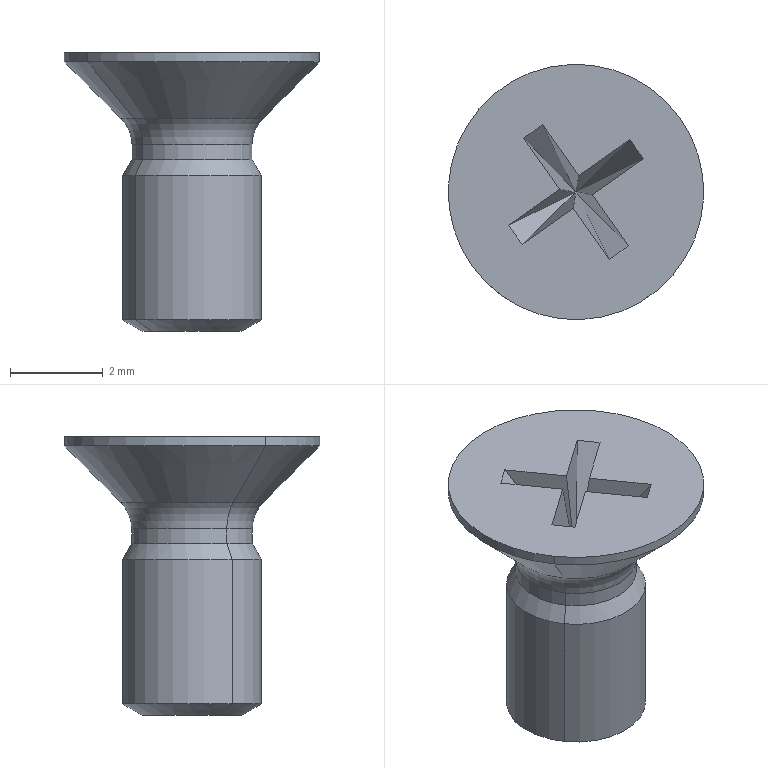Component | SolidWorks | MGL-PACK-03-00Fixture-1_PhillipsCountersunkScrewM3_6[GB_T819.1-2000]-1 | 1 solid | 28 faces | box 5.5 x 5.5 x 6 mm | volume 51 mm3 | plane 14 | cone 6 | cylinder 6 | torus 2 | commonest cylinder face diameters 3 x2 2.598 x2 5.5 x2
STEP:
#1=COLOUR_RGB('',0.7922,0.8196,0.9333);
#2=FILL_AREA_STYLE_COLOUR('',#1);
#3=FILL_AREA_STYLE('',(#2));
#4=SURFACE_STYLE_FILL_AREA(#3);
#5=SURFACE_SIDE_STYLE('',(#4));
#6=SURFACE_STYLE_USAGE(.BOTH.,#5);
#7=PRESENTATION_STYLE_ASSIGNMENT((#6));
#8=CARTESIAN_POINT('',(10.566,1.343,-10.524));
#9=VERTEX_POINT('',#8);
#10=CARTESIAN_POINT('',(10.497,1.295,-10.524));
#11=VERTEX_POINT('',#10);
#12=CARTESIAN_POINT('',(10.531,1.319,-10.524));
#13=DIRECTION('',(-0.,0.,-1.));
#14=DIRECTION('',(0.8166,0.5772,0.));
#15=AXIS2_PLACEMENT_3D('',#12,#13,#14);
#16=CIRCLE('',#15,0.04201);
#17=EDGE_CURVE('',#9,#11,#16,.T.);
#18=ORIENTED_EDGE('',*,*,#17,.F.);
#19=CARTESIAN_POINT('',(10.58,1.353,-10.514));
#20=VERTEX_POINT('',#19);
#21=CARTESIAN_POINT('',(10.58,1.353,-10.514));
#22=DIRECTION('',(0.7091,0.5012,0.4959));
#23=VECTOR('',#22,39.37);
#24=LINE('',#21,#23);
#25=EDGE_CURVE('',#9,#20,#24,.T.);
#26=ORIENTED_EDGE('',*,*,#25,.T.);
#27=CARTESIAN_POINT('',(10.483,1.285,-10.514));
#28=VERTEX_POINT('',#27);
#29=CARTESIAN_POINT('',(10.531,1.319,-10.514));
#30=DIRECTION('',(-0.,0.,-1.));
#31=DIRECTION('',(0.8166,0.5772,0.));
#32=AXIS2_PLACEMENT_3D('',#29,#30,#31);
#33=CIRCLE('',#32,0.05906);
#34=EDGE_CURVE('',#20,#28,#33,.T.);
#35=ORIENTED_EDGE('',*,*,#34,.T.);
#36=CARTESIAN_POINT('',(10.483,1.285,-10.514));
#37=DIRECTION('',(-0.7091,-0.5012,0.4959));
#38=VECTOR('',#37,39.37);
#39=LINE('',#36,#38);
#40=EDGE_CURVE('',#11,#28,#39,.T.);
#41=ORIENTED_EDGE('',*,*,#40,.F.);
#42=EDGE_LOOP('',(#18,#26,#35,#41));
#43=FACE_OUTER_BOUND('',#42,.T.);
#44=CARTESIAN_POINT('',(10.531,1.319,-10.514));
#45=DIRECTION('',(0.,-0.,1.));
#46=DIRECTION('',(-0.8166,-0.5772,0.));
#47=AXIS2_PLACEMENT_3D('',#44,#45,#46);
#48=CONICAL_SURFACE('',#47,0.05906,1.052);
#49=ADVANCED_FACE('',(#43),#48,.T.);
#50=ORIENTED_EDGE('',*,*,#34,.F.);
#51=CARTESIAN_POINT('',(10.58,1.353,-10.392));
#52=VERTEX_POINT('',#51);
#53=CARTESIAN_POINT('',(10.58,1.353,-10.287));
#54=DIRECTION('',(0.,-0.,1.));
#55=VECTOR('',#54,39.37);
#56=LINE('',#53,#55);
#57=EDGE_CURVE('',#20,#52,#56,.T.);
#58=ORIENTED_EDGE('',*,*,#57,.T.);
#59=CARTESIAN_POINT('',(10.483,1.285,-10.392));
#60=VERTEX_POINT('',#59);
#61=CARTESIAN_POINT('',(10.531,1.319,-10.392));
#62=DIRECTION('',(0.,-0.,1.));
#63=DIRECTION('',(-0.8166,-0.5772,0.));
#64=AXIS2_PLACEMENT_3D('',#61,#62,#63);
#65=CIRCLE('',#64,0.05906);
#66=EDGE_CURVE('',#60,#52,#65,.T.);
#67=ORIENTED_EDGE('',*,*,#66,.F.);
#68=CARTESIAN_POINT('',(10.483,1.285,-10.287));
#69=DIRECTION('',(0.,-0.,1.));
#70=VECTOR('',#69,39.37);
#71=LINE('',#68,#70);
#72=EDGE_CURVE('',#28,#60,#71,.T.);
#73=ORIENTED_EDGE('',*,*,#72,.F.);
#74=EDGE_LOOP('',(#50,#58,#67,#73));
#75=FACE_OUTER_BOUND('',#74,.T.);
#76=CARTESIAN_POINT('',(10.531,1.319,-10.287));
#77=DIRECTION('',(0.,-0.,1.));
#78=DIRECTION('',(-0.8166,-0.5772,0.));
#79=AXIS2_PLACEMENT_3D('',#76,#77,#78);
#80=CYLINDRICAL_SURFACE('',#79,0.05906);
#81=ADVANCED_FACE('',(#75),#80,.T.);
#82=CARTESIAN_POINT('',(10.49,1.289,-10.378));
#83=VERTEX_POINT('',#82);
#84=CARTESIAN_POINT('',(10.573,1.348,-10.378));
#85=VERTEX_POINT('',#84);
#86=CARTESIAN_POINT('',(10.531,1.319,-10.378));
#87=DIRECTION('',(0.,-0.,1.));
#88=DIRECTION('',(-0.8166,-0.5772,0.));
#89=AXIS2_PLACEMENT_3D('',#86,#87,#88);
#90=CIRCLE('',#89,0.05114);
#91=EDGE_CURVE('',#83,#85,#90,.T.);
#92=ORIENTED_EDGE('',*,*,#91,.F.);
#93=CARTESIAN_POINT('',(10.483,1.285,-10.392));
#94=DIRECTION('',(-0.4083,-0.2886,-0.866));
#95=VECTOR('',#94,39.37);
#96=LINE('',#93,#95);
#97=EDGE_CURVE('',#83,#60,#96,.T.);
#98=ORIENTED_EDGE('',*,*,#97,.T.);
#99=ORIENTED_EDGE('',*,*,#66,.T.);
#100=CARTESIAN_POINT('',(10.58,1.353,-10.392));
#101=DIRECTION('',(0.4083,0.2886,-0.866));
#102=VECTOR('',#101,39.37);
#103=LINE('',#100,#102);
#104=EDGE_CURVE('',#85,#52,#103,.T.);
#105=ORIENTED_EDGE('',*,*,#104,.F.);
#106=EDGE_LOOP('',(#92,#98,#99,#105));
#107=FACE_OUTER_BOUND('',#106,.T.);
#108=CARTESIAN_POINT('',(10.531,1.319,-10.392));
#109=DIRECTION('',(-0.,0.,-1.));
#110=DIRECTION('',(0.8166,0.5772,0.));
#111=AXIS2_PLACEMENT_3D('',#108,#109,#110);
#112=CONICAL_SURFACE('',#111,0.05906,0.5236);
#113=ADVANCED_FACE('',(#107),#112,.T.);
#114=ORIENTED_EDGE('',*,*,#91,.T.);
#115=CARTESIAN_POINT('',(10.573,1.348,-10.365));
#116=VERTEX_POINT('',#115);
#117=CARTESIAN_POINT('',(10.573,1.348,-10.287));
#118=DIRECTION('',(0.,-0.,1.));
#119=VECTOR('',#118,39.37);
#120=LINE('',#117,#119);
#121=EDGE_CURVE('',#85,#116,#120,.T.);
#122=ORIENTED_EDGE('',*,*,#121,.T.);
#123=CARTESIAN_POINT('',(10.49,1.289,-10.365));
#124=VERTEX_POINT('',#123);
#125=CARTESIAN_POINT('',(10.531,1.319,-10.365));
#126=DIRECTION('',(0.,-0.,1.));
#127=DIRECTION('',(-0.8166,-0.5772,0.));
#128=AXIS2_PLACEMENT_3D('',#125,#126,#127);
#129=CIRCLE('',#128,0.05114);
#130=EDGE_CURVE('',#124,#116,#129,.T.);
#131=ORIENTED_EDGE('',*,*,#130,.F.);
#132=CARTESIAN_POINT('',(10.49,1.289,-10.287));
#133=DIRECTION('',(0.,-0.,1.));
#134=VECTOR('',#133,39.37);
#135=LINE('',#132,#134);
#136=EDGE_CURVE('',#83,#124,#135,.T.);
#137=ORIENTED_EDGE('',*,*,#136,.F.);
#138=EDGE_LOOP('',(#114,#122,#131,#137));
#139=FACE_OUTER_BOUND('',#138,.T.);
#140=CARTESIAN_POINT('',(10.531,1.319,-10.287));
#141=DIRECTION('',(0.,-0.,1.));
#142=DIRECTION('',(-0.8166,-0.5772,0.));
#143=AXIS2_PLACEMENT_3D('',#140,#141,#142);
#144=CYLINDRICAL_SURFACE('',#143,0.05114);
#145=ADVANCED_FACE('',(#139),#144,.T.);
#146=CARTESIAN_POINT('',(10.581,1.354,-10.343));
#147=VERTEX_POINT('',#146);
#148=CARTESIAN_POINT('',(10.482,1.284,-10.343));
#149=VERTEX_POINT('',#148);
#150=CARTESIAN_POINT('',(10.531,1.319,-10.343));
#151=DIRECTION('',(0.,-0.,1.));
#152=DIRECTION('',(-0.8166,-0.5772,0.));
#153=AXIS2_PLACEMENT_3D('',#150,#151,#152);
#154=CIRCLE('',#153,0.06037);
#155=EDGE_CURVE('',#147,#149,#154,.T.);
#156=ORIENTED_EDGE('',*,*,#155,.F.);
#157=CARTESIAN_POINT('',(10.599,1.367,-10.365));
#158=DIRECTION('',(0.5772,-0.8166,-0.));
#159=DIRECTION('',(0.8166,0.5772,0.));
#160=AXIS2_PLACEMENT_3D('',#157,#158,#159);
#161=CIRCLE('',#160,0.0315);
#162=EDGE_CURVE('',#147,#116,#161,.T.);
#163=ORIENTED_EDGE('',*,*,#162,.T.);
#164=CARTESIAN_POINT('',(10.531,1.319,-10.365));
#165=DIRECTION('',(0.,-0.,1.));
#166=DIRECTION('',(-0.8166,-0.5772,0.));
#167=AXIS2_PLACEMENT_3D('',#164,#165,#166);
#168=CIRCLE('',#167,0.05114);
#169=EDGE_CURVE('',#116,#124,#168,.T.);
#170=ORIENTED_EDGE('',*,*,#169,.T.);
#171=CARTESIAN_POINT('',(10.464,1.271,-10.365));
#172=DIRECTION('',(-0.5772,0.8166,0.));
#173=DIRECTION('',(-0.8166,-0.5772,0.));
#174=AXIS2_PLACEMENT_3D('',#171,#172,#173);
#175=CIRCLE('',#174,0.0315);
#176=EDGE_CURVE('',#149,#124,#175,.T.);
#177=ORIENTED_EDGE('',*,*,#176,.F.);
#178=EDGE_LOOP('',(#156,#163,#170,#177));
#179=FACE_OUTER_BOUND('',#178,.T.);
#180=CARTESIAN_POINT('',(10.531,1.319,-10.365));
#181=DIRECTION('',(0.,-0.,1.));
#182=DIRECTION('',(-0.8166,-0.5772,-0.));
#183=AXIS2_PLACEMENT_3D('',#180,#181,#182);
#184=TOROIDAL_SURFACE('',#183,0.08264,0.0315);
#185=ADVANCED_FACE('',(#179),#184,.F.);
#186=CARTESIAN_POINT('',(10.531,1.319,-10.343));
#187=DIRECTION('',(0.,-0.,1.));
#188=DIRECTION('',(-0.8166,-0.5772,0.));
#189=AXIS2_PLACEMENT_3D('',#186,#187,#188);
#190=CIRCLE('',#189,0.06037);
#191=EDGE_CURVE('',#149,#147,#190,.T.);
#192=ORIENTED_EDGE('',*,*,#191,.T.);
#193=CARTESIAN_POINT('',(10.62,1.381,-10.295));
#194=VERTEX_POINT('',#193);
#195=CARTESIAN_POINT('',(10.581,1.354,-10.343));
#196=DIRECTION('',(0.5774,0.4081,0.7071));
#197=VECTOR('',#196,39.37);
#198=LINE('',#195,#197);
#199=EDGE_CURVE('',#147,#194,#198,.T.);
#200=ORIENTED_EDGE('',*,*,#199,.T.);
#201=CARTESIAN_POINT('',(10.443,1.256,-10.295));
#202=VERTEX_POINT('',#201);
#203=CARTESIAN_POINT('',(10.531,1.319,-10.295));
#204=DIRECTION('',(0.,-0.,1.));
#205=DIRECTION('',(-0.8166,-0.5772,0.));
#206=AXIS2_PLACEMENT_3D('',#203,#204,#205);
#207=CIRCLE('',#206,0.1083);
#208=EDGE_CURVE('',#202,#194,#207,.T.);
#209=ORIENTED_EDGE('',*,*,#208,.F.);
#210=CARTESIAN_POINT('',(10.482,1.284,-10.343));
#211=DIRECTION('',(-0.5774,-0.4081,0.7071));
#212=VECTOR('',#211,39.37);
#213=LINE('',#210,#212);
#214=EDGE_CURVE('',#149,#202,#213,.T.);
#215=ORIENTED_EDGE('',*,*,#214,.F.);
#216=EDGE_LOOP('',(#192,#200,#209,#215));
#217=FACE_OUTER_BOUND('',#216,.T.);
#218=CARTESIAN_POINT('',(10.531,1.319,-10.343));
#219=DIRECTION('',(0.,-0.,1.));
#220=DIRECTION('',(-0.8166,-0.5772,0.));
#221=AXIS2_PLACEMENT_3D('',#218,#219,#220);
#222=CONICAL_SURFACE('',#221,0.06037,0.7854);
#223=ADVANCED_FACE('',(#217),#222,.T.);
#224=ORIENTED_EDGE('',*,*,#208,.T.);
#225=CARTESIAN_POINT('',(10.62,1.381,-10.287));
#226=VERTEX_POINT('',#225);
#227=CARTESIAN_POINT('',(10.62,1.381,-10.287));
#228=DIRECTION('',(0.,-0.,1.));
#229=VECTOR('',#228,39.37);
#230=LINE('',#227,#229);
#231=EDGE_CURVE('',#194,#226,#230,.T.);
#232=ORIENTED_EDGE('',*,*,#231,.T.);
#233=CARTESIAN_POINT('',(10.443,1.256,-10.287));
#234=VERTEX_POINT('',#233);
#235=CARTESIAN_POINT('',(10.531,1.319,-10.287));
#236=DIRECTION('',(0.,-0.,1.));
#237=DIRECTION('',(-0.8166,-0.5772,0.));
#238=AXIS2_PLACEMENT_3D('',#235,#236,#237);
#239=CIRCLE('',#238,0.1083);
#240=EDGE_CURVE('',#234,#226,#239,.T.);
#241=ORIENTED_EDGE('',*,*,#240,.F.);
#242=CARTESIAN_POINT('',(10.443,1.256,-10.287));
#243=DIRECTION('',(0.,-0.,1.));
#244=VECTOR('',#243,39.37);
#245=LINE('',#242,#244);
#246=EDGE_CURVE('',#202,#234,#245,.T.);
#247=ORIENTED_EDGE('',*,*,#246,.F.);
#248=EDGE_LOOP('',(#224,#232,#241,#247));
#249=FACE_OUTER_BOUND('',#248,.T.);
#250=CARTESIAN_POINT('',(10.531,1.319,-10.287));
#251=DIRECTION('',(0.,-0.,1.));
#252=DIRECTION('',(-0.8166,-0.5772,0.));
#253=AXIS2_PLACEMENT_3D('',#250,#251,#252);
#254=CYLINDRICAL_SURFACE('',#253,0.1083);
#255=ADVANCED_FACE('',(#249),#254,.T.);
#256=ORIENTED_EDGE('',*,*,#240,.T.);
#257=CARTESIAN_POINT('',(10.531,1.319,-10.287));
#258=DIRECTION('',(0.,-0.,1.));
#259=DIRECTION('',(-0.8166,-0.5772,0.));
#260=AXIS2_PLACEMENT_3D('',#257,#258,#259);
#261=CIRCLE('',#260,0.1083);
#262=EDGE_CURVE('',#226,#234,#261,.T.);
#263=ORIENTED_EDGE('',*,*,#262,.T.);
#264=EDGE_LOOP('',(#256,#263));
#265=FACE_OUTER_BOUND('',#264,.T.);
#266=CARTESIAN_POINT('',(10.529,1.305,-10.287));
#267=VERTEX_POINT('',#266);
#268=CARTESIAN_POINT('',(10.56,1.262,-10.287));
#269=VERTEX_POINT('',#268);
#270=CARTESIAN_POINT('',(10.56,1.262,-10.287));
#271=DIRECTION('',(0.5772,-0.8166,-0.));
#272=VECTOR('',#271,39.37);
#273=LINE('',#270,#272);
#274=EDGE_CURVE('',#267,#269,#273,.T.);
#275=ORIENTED_EDGE('',*,*,#274,.F.);
#276=CARTESIAN_POINT('',(10.486,1.275,-10.287));
#277=VERTEX_POINT('',#276);
#278=CARTESIAN_POINT('',(10.589,1.347,-10.287));
#279=DIRECTION('',(0.8166,0.5772,0.));
#280=VECTOR('',#279,39.37);
#281=LINE('',#278,#280);
#282=EDGE_CURVE('',#277,#267,#281,.T.);
#283=ORIENTED_EDGE('',*,*,#282,.F.);
#284=CARTESIAN_POINT('',(10.474,1.291,-10.287));
#285=VERTEX_POINT('',#284);
#286=CARTESIAN_POINT('',(10.486,1.275,-10.287));
#287=DIRECTION('',(0.5772,-0.8166,-0.));
#288=VECTOR('',#287,39.37);
#289=LINE('',#286,#288);
#290=EDGE_CURVE('',#285,#277,#289,.T.);
#291=ORIENTED_EDGE('',*,*,#290,.F.);
#292=CARTESIAN_POINT('',(10.518,1.321,-10.287));
#293=VERTEX_POINT('',#292);
#294=CARTESIAN_POINT('',(10.577,1.363,-10.287));
#295=DIRECTION('',(-0.8166,-0.5772,-0.));
#296=VECTOR('',#295,39.37);
#297=LINE('',#294,#296);
#298=EDGE_CURVE('',#293,#285,#297,.T.);
#299=ORIENTED_EDGE('',*,*,#298,.F.);
#300=CARTESIAN_POINT('',(10.487,1.365,-10.287));
#301=VERTEX_POINT('',#300);
#302=CARTESIAN_POINT('',(10.56,1.262,-10.287));
#303=DIRECTION('',(0.5772,-0.8166,-0.));
#304=VECTOR('',#303,39.37);
#305=LINE('',#302,#304);
#306=EDGE_CURVE('',#301,#293,#305,.T.);
#307=ORIENTED_EDGE('',*,*,#306,.F.);
#308=CARTESIAN_POINT('',(10.503,1.376,-10.287));
#309=VERTEX_POINT('',#308);
#310=CARTESIAN_POINT('',(10.487,1.365,-10.287));
#311=DIRECTION('',(-0.8166,-0.5772,-0.));
#312=VECTOR('',#311,39.37);
#313=LINE('',#310,#312);
#314=EDGE_CURVE('',#309,#301,#313,.T.);
#315=ORIENTED_EDGE('',*,*,#314,.F.);
#316=CARTESIAN_POINT('',(10.534,1.333,-10.287));
#317=VERTEX_POINT('',#316);
#318=CARTESIAN_POINT('',(10.576,1.273,-10.287));
#319=DIRECTION('',(-0.5772,0.8166,0.));
#320=VECTOR('',#319,39.37);
#321=LINE('',#318,#320);
#322=EDGE_CURVE('',#317,#309,#321,.T.);
#323=ORIENTED_EDGE('',*,*,#322,.F.);
#324=CARTESIAN_POINT('',(10.577,1.363,-10.287));
#325=VERTEX_POINT('',#324);
#326=CARTESIAN_POINT('',(10.577,1.363,-10.287));
#327=DIRECTION('',(-0.8166,-0.5772,-0.));
#328=VECTOR('',#327,39.37);
#329=LINE('',#326,#328);
#330=EDGE_CURVE('',#325,#317,#329,.T.);
#331=ORIENTED_EDGE('',*,*,#330,.F.);
#332=CARTESIAN_POINT('',(10.589,1.347,-10.287));
#333=VERTEX_POINT('',#332);
#334=CARTESIAN_POINT('',(10.589,1.347,-10.287));
#335=DIRECTION('',(-0.5772,0.8166,0.));
#336=VECTOR('',#335,39.37);
#337=LINE('',#334,#336);
#338=EDGE_CURVE('',#333,#325,#337,.T.);
#339=ORIENTED_EDGE('',*,*,#338,.F.);
#340=CARTESIAN_POINT('',(10.545,1.317,-10.287));
#341=VERTEX_POINT('',#340);
#342=CARTESIAN_POINT('',(10.589,1.347,-10.287));
#343=DIRECTION('',(0.8166,0.5772,0.));
#344=VECTOR('',#343,39.37);
#345=LINE('',#342,#344);
#346=EDGE_CURVE('',#341,#333,#345,.T.);
#347=ORIENTED_EDGE('',*,*,#346,.F.);
#348=CARTESIAN_POINT('',(10.576,1.273,-10.287));
#349=VERTEX_POINT('',#348);
#350=CARTESIAN_POINT('',(10.576,1.273,-10.287));
#351=DIRECTION('',(-0.5772,0.8166,0.));
#352=VECTOR('',#351,39.37);
#353=LINE('',#350,#352);
#354=EDGE_CURVE('',#349,#341,#353,.T.);
#355=ORIENTED_EDGE('',*,*,#354,.F.);
#356=CARTESIAN_POINT('',(10.56,1.262,-10.287));
#357=DIRECTION('',(0.8166,0.5772,0.));
#358=VECTOR('',#357,39.37);
#359=LINE('',#356,#358);
#360=EDGE_CURVE('',#269,#349,#359,.T.);
#361=ORIENTED_EDGE('',*,*,#360,.F.);
#362=EDGE_LOOP('',(#275,#283,#291,#299,#307,#315,#323,#331,#339,#347,#355,#361));
#363=FACE_BOUND('',#362,.T.);
#364=CARTESIAN_POINT('',(10.531,1.319,-10.287));
#365=DIRECTION('',(-0.,0.,-1.));
#366=DIRECTION('',(0.8166,0.5772,0.));
#367=AXIS2_PLACEMENT_3D('',#364,#365,#366);
#368=PLANE('',#367);
#369=ADVANCED_FACE('',(#265,#363),#368,.F.);
#370=ORIENTED_EDGE('',*,*,#282,.T.);
#371=CARTESIAN_POINT('',(10.531,1.319,-10.37));
#372=VERTEX_POINT('',#371);
#373=CARTESIAN_POINT('',(10.531,1.319,-10.37));
#374=DIRECTION('',(0.02811,0.1636,-0.9861));
#375=VECTOR('',#374,39.37);
#376=LINE('',#373,#375);
#377=EDGE_CURVE('',#267,#372,#376,.T.);
#378=ORIENTED_EDGE('',*,*,#377,.T.);
#379=CARTESIAN_POINT('',(10.486,1.275,-10.287));
#380=DIRECTION('',(0.4383,0.4252,-0.7919));
#381=VECTOR('',#380,39.37);
#382=LINE('',#379,#381);
#383=EDGE_CURVE('',#277,#372,#382,.T.);
#384=ORIENTED_EDGE('',*,*,#383,.F.);
#385=EDGE_LOOP('',(#370,#378,#384));
#386=FACE_OUTER_BOUND('',#385,.T.);
#387=CARTESIAN_POINT('',(10.531,1.319,-10.37));
#388=DIRECTION('',(-0.5731,0.8109,0.1182));
#389=DIRECTION('',(-0.06823,0.09653,-0.993));
#390=AXIS2_PLACEMENT_3D('',#387,#388,#389);
#391=PLANE('',#390);
#392=ADVANCED_FACE('',(#386),#391,.T.);
#393=CARTESIAN_POINT('',(10.589,1.347,-10.287));
#394=DIRECTION('',(-0.5471,-0.2713,-0.7919));
#395=VECTOR('',#394,39.37);
#396=LINE('',#393,#395);
#397=EDGE_CURVE('',#333,#372,#396,.T.);
#398=ORIENTED_EDGE('',*,*,#397,.T.);
#399=CARTESIAN_POINT('',(10.531,1.319,-10.37));
#400=DIRECTION('',(0.1636,-0.02811,0.9861));
#401=VECTOR('',#400,39.37);
#402=LINE('',#399,#401);
#403=EDGE_CURVE('',#372,#341,#402,.T.);
#404=ORIENTED_EDGE('',*,*,#403,.T.);
#405=ORIENTED_EDGE('',*,*,#346,.T.);
#406=EDGE_LOOP('',(#398,#404,#405));
#407=FACE_OUTER_BOUND('',#406,.T.);
#408=CARTESIAN_POINT('',(10.531,1.319,-10.37));
#409=DIRECTION('',(-0.5731,0.8109,0.1182));
#410=DIRECTION('',(-0.06823,0.09653,-0.993));
#411=AXIS2_PLACEMENT_3D('',#408,#409,#410);
#412=PLANE('',#411);
#413=ADVANCED_FACE('',(#407),#412,.T.);
#414=CARTESIAN_POINT('',(10.474,1.291,-10.287));
#415=DIRECTION('',(0.5471,0.2713,-0.7919));
#416=VECTOR('',#415,39.37);
#417=LINE('',#414,#416);
#418=EDGE_CURVE('',#285,#372,#417,.T.);
#419=ORIENTED_EDGE('',*,*,#418,.T.);
#420=CARTESIAN_POINT('',(10.531,1.319,-10.37));
#421=DIRECTION('',(-0.1636,0.02811,0.9861));
#422=VECTOR('',#421,39.37);
#423=LINE('',#420,#422);
#424=EDGE_CURVE('',#372,#293,#423,.T.);
#425=ORIENTED_EDGE('',*,*,#424,.T.);
#426=ORIENTED_EDGE('',*,*,#298,.T.);
#427=EDGE_LOOP('',(#419,#425,#426));
#428=FACE_OUTER_BOUND('',#427,.T.);
#429=CARTESIAN_POINT('',(10.531,1.319,-10.37));
#430=DIRECTION('',(0.5731,-0.8109,0.1182));
#431=DIRECTION('',(-0.06823,0.09653,0.993));
#432=AXIS2_PLACEMENT_3D('',#429,#430,#431);
#433=PLANE('',#432);
#434=ADVANCED_FACE('',(#428),#433,.T.);
#435=ORIENTED_EDGE('',*,*,#330,.T.);
#436=CARTESIAN_POINT('',(10.531,1.319,-10.37));
#437=DIRECTION('',(-0.02811,-0.1636,-0.9861));
#438=VECTOR('',#437,39.37);
#439=LINE('',#436,#438);
#440=EDGE_CURVE('',#317,#372,#439,.T.);
#441=ORIENTED_EDGE('',*,*,#440,.T.);
#442=CARTESIAN_POINT('',(10.577,1.363,-10.287));
#443=DIRECTION('',(-0.4383,-0.4252,-0.7919));
#444=VECTOR('',#443,39.37);
#445=LINE('',#442,#444);
#446=EDGE_CURVE('',#325,#372,#445,.T.);
#447=ORIENTED_EDGE('',*,*,#446,.F.);
#448=EDGE_LOOP('',(#435,#441,#447));
#449=FACE_OUTER_BOUND('',#448,.T.);
#450=CARTESIAN_POINT('',(10.531,1.319,-10.37));
#451=DIRECTION('',(0.5731,-0.8109,0.1182));
#452=DIRECTION('',(-0.06823,0.09653,0.993));
#453=AXIS2_PLACEMENT_3D('',#450,#451,#452);
#454=PLANE('',#453);
#455=ADVANCED_FACE('',(#449),#454,.T.);
#456=ORIENTED_EDGE('',*,*,#231,.F.);
#457=CARTESIAN_POINT('',(10.531,1.319,-10.295));
#458=DIRECTION('',(0.,-0.,1.));
#459=DIRECTION('',(-0.8166,-0.5772,0.));
#460=AXIS2_PLACEMENT_3D('',#457,#458,#459);
#461=CIRCLE('',#460,0.1083);
#462=EDGE_CURVE('',#194,#202,#461,.T.);
#463=ORIENTED_EDGE('',*,*,#462,.T.);
#464=ORIENTED_EDGE('',*,*,#246,.T.);
#465=ORIENTED_EDGE('',*,*,#262,.F.);
#466=EDGE_LOOP('',(#456,#463,#464,#465));
#467=FACE_OUTER_BOUND('',#466,.T.);
#468=CARTESIAN_POINT('',(10.531,1.319,-10.287));
#469=DIRECTION('',(0.,-0.,1.));
#470=DIRECTION('',(-0.8166,-0.5772,0.));
#471=AXIS2_PLACEMENT_3D('',#468,#469,#470);
#472=CYLINDRICAL_SURFACE('',#471,0.1083);
#473=ADVANCED_FACE('',(#467),#472,.T.);
#474=ORIENTED_EDGE('',*,*,#199,.F.);
#475=ORIENTED_EDGE('',*,*,#155,.T.);
#476=ORIENTED_EDGE('',*,*,#214,.T.);
#477=ORIENTED_EDGE('',*,*,#462,.F.);
#478=EDGE_LOOP('',(#474,#475,#476,#477));
#479=FACE_OUTER_BOUND('',#478,.T.);
#480=CARTESIAN_POINT('',(10.531,1.319,-10.343));
#481=DIRECTION('',(0.,-0.,1.));
#482=DIRECTION('',(-0.8166,-0.5772,0.));
#483=AXIS2_PLACEMENT_3D('',#480,#481,#482);
#484=CONICAL_SURFACE('',#483,0.06037,0.7854);
#485=ADVANCED_FACE('',(#479),#484,.T.);
#486=ORIENTED_EDGE('',*,*,#162,.F.);
#487=ORIENTED_EDGE('',*,*,#191,.F.);
#488=ORIENTED_EDGE('',*,*,#176,.T.);
#489=ORIENTED_EDGE('',*,*,#130,.T.);
#490=EDGE_LOOP('',(#486,#487,#488,#489));
#491=FACE_OUTER_BOUND('',#490,.T.);
#492=CARTESIAN_POINT('',(10.531,1.319,-10.365));
#493=DIRECTION('',(0.,-0.,1.));
#494=DIRECTION('',(-0.8166,-0.5772,-0.));
#495=AXIS2_PLACEMENT_3D('',#492,#493,#494);
#496=TOROIDAL_SURFACE('',#495,0.08264,0.0315);
#497=ADVANCED_FACE('',(#491),#496,.F.);
#498=ORIENTED_EDGE('',*,*,#121,.F.);
#499=CARTESIAN_POINT('',(10.531,1.319,-10.378));
#500=DIRECTION('',(0.,-0.,1.));
#501=DIRECTION('',(-0.8166,-0.5772,0.));
#502=AXIS2_PLACEMENT_3D('',#499,#500,#501);
#503=CIRCLE('',#502,0.05114);
#504=EDGE_CURVE('',#85,#83,#503,.T.);
#505=ORIENTED_EDGE('',*,*,#504,.T.);
#506=ORIENTED_EDGE('',*,*,#136,.T.);
#507=ORIENTED_EDGE('',*,*,#169,.F.);
#508=EDGE_LOOP('',(#498,#505,#506,#507));
#509=FACE_OUTER_BOUND('',#508,.T.);
#510=CARTESIAN_POINT('',(10.531,1.319,-10.287));
#511=DIRECTION('',(0.,-0.,1.));
#512=DIRECTION('',(-0.8166,-0.5772,0.));
#513=AXIS2_PLACEMENT_3D('',#510,#511,#512);
#514=CYLINDRICAL_SURFACE('',#513,0.05114);
#515=ADVANCED_FACE('',(#509),#514,.T.);
#516=ORIENTED_EDGE('',*,*,#97,.F.);
#517=ORIENTED_EDGE('',*,*,#504,.F.);
#518=ORIENTED_EDGE('',*,*,#104,.T.);
#519=CARTESIAN_POINT('',(10.531,1.319,-10.392));
#520=DIRECTION('',(0.,-0.,1.));
#521=DIRECTION('',(-0.8166,-0.5772,0.));
#522=AXIS2_PLACEMENT_3D('',#519,#520,#521);
#523=CIRCLE('',#522,0.05906);
#524=EDGE_CURVE('',#52,#60,#523,.T.);
#525=ORIENTED_EDGE('',*,*,#524,.T.);
#526=EDGE_LOOP('',(#516,#517,#518,#525));
#527=FACE_OUTER_BOUND('',#526,.T.);
#528=CARTESIAN_POINT('',(10.531,1.319,-10.392));
#529=DIRECTION('',(-0.,0.,-1.));
#530=DIRECTION('',(0.8166,0.5772,0.));
#531=AXIS2_PLACEMENT_3D('',#528,#529,#530);
#532=CONICAL_SURFACE('',#531,0.05906,0.5236);
#533=ADVANCED_FACE('',(#527),#532,.T.);
#534=ORIENTED_EDGE('',*,*,#57,.F.);
#535=CARTESIAN_POINT('',(10.531,1.319,-10.514));
#536=DIRECTION('',(-0.,0.,-1.));
#537=DIRECTION('',(0.8166,0.5772,0.));
#538=AXIS2_PLACEMENT_3D('',#535,#536,#537);
#539=CIRCLE('',#538,0.05906);
#540=EDGE_CURVE('',#28,#20,#539,.T.);
#541=ORIENTED_EDGE('',*,*,#540,.F.);
#542=ORIENTED_EDGE('',*,*,#72,.T.);
#543=ORIENTED_EDGE('',*,*,#524,.F.);
#544=EDGE_LOOP('',(#534,#541,#542,#543));
#545=FACE_OUTER_BOUND('',#544,.T.);
#546=CARTESIAN_POINT('',(10.531,1.319,-10.287));
#547=DIRECTION('',(0.,-0.,1.));
#548=DIRECTION('',(-0.8166,-0.5772,0.));
#549=AXIS2_PLACEMENT_3D('',#546,#547,#548);
#550=CYLINDRICAL_SURFACE('',#549,0.05906);
#551=ADVANCED_FACE('',(#545),#550,.T.);
#552=ORIENTED_EDGE('',*,*,#25,.F.);
#553=CARTESIAN_POINT('',(10.531,1.319,-10.524));
#554=DIRECTION('',(-0.,0.,-1.));
#555=DIRECTION('',(0.8166,0.5772,0.));
#556=AXIS2_PLACEMENT_3D('',#553,#554,#555);
#557=CIRCLE('',#556,0.04201);
#558=EDGE_CURVE('',#11,#9,#557,.T.);
#559=ORIENTED_EDGE('',*,*,#558,.F.);
#560=ORIENTED_EDGE('',*,*,#40,.T.);
#561=ORIENTED_EDGE('',*,*,#540,.T.);
#562=EDGE_LOOP('',(#552,#559,#560,#561));
#563=FACE_OUTER_BOUND('',#562,.T.);
#564=CARTESIAN_POINT('',(10.531,1.319,-10.514));
#565=DIRECTION('',(0.,-0.,1.));
#566=DIRECTION('',(-0.8166,-0.5772,0.));
#567=AXIS2_PLACEMENT_3D('',#564,#565,#566);
#568=CONICAL_SURFACE('',#567,0.05906,1.052);
#569=ADVANCED_FACE('',(#563),#568,.T.);
#570=ORIENTED_EDGE('',*,*,#558,.T.);
#571=ORIENTED_EDGE('',*,*,#17,.T.);
#572=EDGE_LOOP('',(#570,#571));
#573=FACE_OUTER_BOUND('',#572,.T.);
#574=CARTESIAN_POINT('',(10.566,1.271,-10.524));
#575=DIRECTION('',(0.,-0.,1.));
#576=DIRECTION('',(-0.8166,-0.5772,-0.));
#577=AXIS2_PLACEMENT_3D('',#574,#575,#576);
#578=PLANE('',#577);
#579=ADVANCED_FACE('',(#573),#578,.F.);
#580=ORIENTED_EDGE('',*,*,#397,.F.);
#581=ORIENTED_EDGE('',*,*,#338,.T.);
#582=ORIENTED_EDGE('',*,*,#446,.T.);
#583=EDGE_LOOP('',(#580,#581,#582));
#584=FACE_OUTER_BOUND('',#583,.T.);
#585=CARTESIAN_POINT('',(10.589,1.347,-10.287));
#586=DIRECTION('',(0.6496,0.4591,-0.606));
#587=DIRECTION('',(0.4949,0.3498,0.7954));
#588=AXIS2_PLACEMENT_3D('',#585,#586,#587);
#589=PLANE('',#588);
#590=ADVANCED_FACE('',(#584),#589,.F.);
#591=ORIENTED_EDGE('',*,*,#418,.F.);
#592=ORIENTED_EDGE('',*,*,#290,.T.);
#593=ORIENTED_EDGE('',*,*,#383,.T.);
#594=EDGE_LOOP('',(#591,#592,#593));
#595=FACE_OUTER_BOUND('',#594,.T.);
#596=CARTESIAN_POINT('',(10.474,1.291,-10.287));
#597=DIRECTION('',(-0.6496,-0.4591,-0.606));
#598=DIRECTION('',(0.4949,0.3498,-0.7954));
#599=AXIS2_PLACEMENT_3D('',#596,#597,#598);
#600=PLANE('',#599);
#601=ADVANCED_FACE('',(#595),#600,.F.);
#602=CARTESIAN_POINT('',(10.487,1.365,-10.287));
#603=DIRECTION('',(0.4252,-0.4383,-0.7919));
#604=VECTOR('',#603,39.37);
#605=LINE('',#602,#604);
#606=EDGE_CURVE('',#301,#372,#605,.T.);
#607=ORIENTED_EDGE('',*,*,#606,.F.);
#608=ORIENTED_EDGE('',*,*,#306,.T.);
#609=ORIENTED_EDGE('',*,*,#424,.F.);
#610=EDGE_LOOP('',(#607,#608,#609));
#611=FACE_OUTER_BOUND('',#610,.T.);
#612=CARTESIAN_POINT('',(10.531,1.319,-10.37));
#613=DIRECTION('',(0.8109,0.5731,0.1182));
#614=DIRECTION('',(0.09653,0.06823,-0.993));
#615=AXIS2_PLACEMENT_3D('',#612,#613,#614);
#616=PLANE('',#615);
#617=ADVANCED_FACE('',(#611),#616,.T.);
#618=ORIENTED_EDGE('',*,*,#322,.T.);
#619=CARTESIAN_POINT('',(10.503,1.376,-10.287));
#620=DIRECTION('',(0.2713,-0.5471,-0.7919));
#621=VECTOR('',#620,39.37);
#622=LINE('',#619,#621);
#623=EDGE_CURVE('',#309,#372,#622,.T.);
#624=ORIENTED_EDGE('',*,*,#623,.T.);
#625=ORIENTED_EDGE('',*,*,#440,.F.);
#626=EDGE_LOOP('',(#618,#624,#625));
#627=FACE_OUTER_BOUND('',#626,.T.);
#628=CARTESIAN_POINT('',(10.531,1.319,-10.37));
#629=DIRECTION('',(-0.8109,-0.5731,0.1182));
#630=DIRECTION('',(0.09653,0.06823,0.993));
#631=AXIS2_PLACEMENT_3D('',#628,#629,#630);
#632=PLANE('',#631);
#633=ADVANCED_FACE('',(#627),#632,.T.);
#634=ORIENTED_EDGE('',*,*,#623,.F.);
#635=ORIENTED_EDGE('',*,*,#314,.T.);
#636=ORIENTED_EDGE('',*,*,#606,.T.);
#637=EDGE_LOOP('',(#634,#635,#636));
#638=FACE_OUTER_BOUND('',#637,.T.);
#639=CARTESIAN_POINT('',(10.503,1.376,-10.287));
#640=DIRECTION('',(-0.4591,0.6496,-0.606));
#641=DIRECTION('',(0.3498,-0.4949,-0.7954));
#642=AXIS2_PLACEMENT_3D('',#639,#640,#641);
#643=PLANE('',#642);
#644=ADVANCED_FACE('',(#638),#643,.F.);
#645=ORIENTED_EDGE('',*,*,#274,.T.);
#646=CARTESIAN_POINT('',(10.56,1.262,-10.287));
#647=DIRECTION('',(-0.2713,0.5471,-0.7919));
#648=VECTOR('',#647,39.37);
#649=LINE('',#646,#648);
#650=EDGE_CURVE('',#269,#372,#649,.T.);
#651=ORIENTED_EDGE('',*,*,#650,.T.);
#652=ORIENTED_EDGE('',*,*,#377,.F.);
#653=EDGE_LOOP('',(#645,#651,#652));
#654=FACE_OUTER_BOUND('',#653,.T.);
#655=CARTESIAN_POINT('',(10.531,1.319,-10.37));
#656=DIRECTION('',(0.8109,0.5731,0.1182));
#657=DIRECTION('',(0.09653,0.06823,-0.993));
#658=AXIS2_PLACEMENT_3D('',#655,#656,#657);
#659=PLANE('',#658);
#660=ADVANCED_FACE('',(#654),#659,.T.);
#661=CARTESIAN_POINT('',(10.576,1.273,-10.287));
#662=DIRECTION('',(-0.4252,0.4383,-0.7919));
#663=VECTOR('',#662,39.37);
#664=LINE('',#661,#663);
#665=EDGE_CURVE('',#349,#372,#664,.T.);
#666=ORIENTED_EDGE('',*,*,#665,.F.);
#667=ORIENTED_EDGE('',*,*,#354,.T.);
#668=ORIENTED_EDGE('',*,*,#403,.F.);
#669=EDGE_LOOP('',(#666,#667,#668));
#670=FACE_OUTER_BOUND('',#669,.T.);
#671=CARTESIAN_POINT('',(10.531,1.319,-10.37));
#672=DIRECTION('',(-0.8109,-0.5731,0.1182));
#673=DIRECTION('',(0.09653,0.06823,0.993));
#674=AXIS2_PLACEMENT_3D('',#671,#672,#673);
#675=PLANE('',#674);
#676=ADVANCED_FACE('',(#670),#675,.T.);
#677=ORIENTED_EDGE('',*,*,#650,.F.);
#678=ORIENTED_EDGE('',*,*,#360,.T.);
#679=ORIENTED_EDGE('',*,*,#665,.T.);
#680=EDGE_LOOP('',(#677,#678,#679));
#681=FACE_OUTER_BOUND('',#680,.T.);
#682=CARTESIAN_POINT('',(10.56,1.262,-10.287));
#683=DIRECTION('',(0.4591,-0.6496,-0.606));
#684=DIRECTION('',(0.3498,-0.4949,0.7954));
#685=AXIS2_PLACEMENT_3D('',#682,#683,#684);
#686=PLANE('',#685);
#687=ADVANCED_FACE('',(#681),#686,.F.);
#688=CLOSED_SHELL('',(#49,#81,#113,#145,#185,#223,#255,#369,#392,#413,#434,#455,#473,#485,#497,#515,#533,#551,#569,#579,#590,#601,#617,#633,#644,#660,#676,#687));
#689=MANIFOLD_SOLID_BREP('',#688);
#690=STYLED_ITEM('',(#7),#689);
#691=PRESENTATION_LAYER_ASSIGNMENT('','',(#690));
#692=(LENGTH_UNIT()NAMED_UNIT(*)SI_UNIT($,.METRE.));
#693=LENGTH_MEASURE_WITH_UNIT(LENGTH_MEASURE(0.0254),#692);
#694=DIMENSIONAL_EXPONENTS(1.,0.,0.,0.,0.,0.,0.);
#695=(CONVERSION_BASED_UNIT('',#693)LENGTH_UNIT()NAMED_UNIT(#694));
#696=UNCERTAINTY_MEASURE_WITH_UNIT(LENGTH_MEASURE(0.00001),#695,'','');
#697=(NAMED_UNIT(*)PLANE_ANGLE_UNIT()SI_UNIT($,.RADIAN.));
#698=(NAMED_UNIT(*)SI_UNIT($,.STERADIAN.)SOLID_ANGLE_UNIT());
#699=(GEOMETRIC_REPRESENTATION_CONTEXT(3)GLOBAL_UNCERTAINTY_ASSIGNED_CONTEXT((#696))GLOBAL_UNIT_ASSIGNED_CONTEXT((#695,#697,#698))REPRESENTATION_CONTEXT('',''));
#700=MECHANICAL_DESIGN_GEOMETRIC_PRESENTATION_REPRESENTATION('',(#690),#699);
#701=CARTESIAN_POINT('',(0.,0.,0.));
#702=DIRECTION('',(0.,0.,1.));
#703=DIRECTION('',(1.,0.,0.));
#704=AXIS2_PLACEMENT_3D('',#701,#702,#703);
#705=(LENGTH_UNIT()NAMED_UNIT(*)SI_UNIT($,.METRE.));
#706=LENGTH_MEASURE_WITH_UNIT(LENGTH_MEASURE(0.0254),#705);
#707=DIMENSIONAL_EXPONENTS(1.,0.,0.,0.,0.,0.,0.);
#708=(CONVERSION_BASED_UNIT('',#706)LENGTH_UNIT()NAMED_UNIT(#707));
#709=UNCERTAINTY_MEASURE_WITH_UNIT(LENGTH_MEASURE(0.00001),#708,'','');
#710=(NAMED_UNIT(*)PLANE_ANGLE_UNIT()SI_UNIT($,.RADIAN.));
#711=(NAMED_UNIT(*)SI_UNIT($,.STERADIAN.)SOLID_ANGLE_UNIT());
#712=(GEOMETRIC_REPRESENTATION_CONTEXT(3)GLOBAL_UNCERTAINTY_ASSIGNED_CONTEXT((#709))GLOBAL_UNIT_ASSIGNED_CONTEXT((#708,#710,#711))REPRESENTATION_CONTEXT('',''));
#713=ADVANCED_BREP_SHAPE_REPRESENTATION('',(#689,#704),#712);